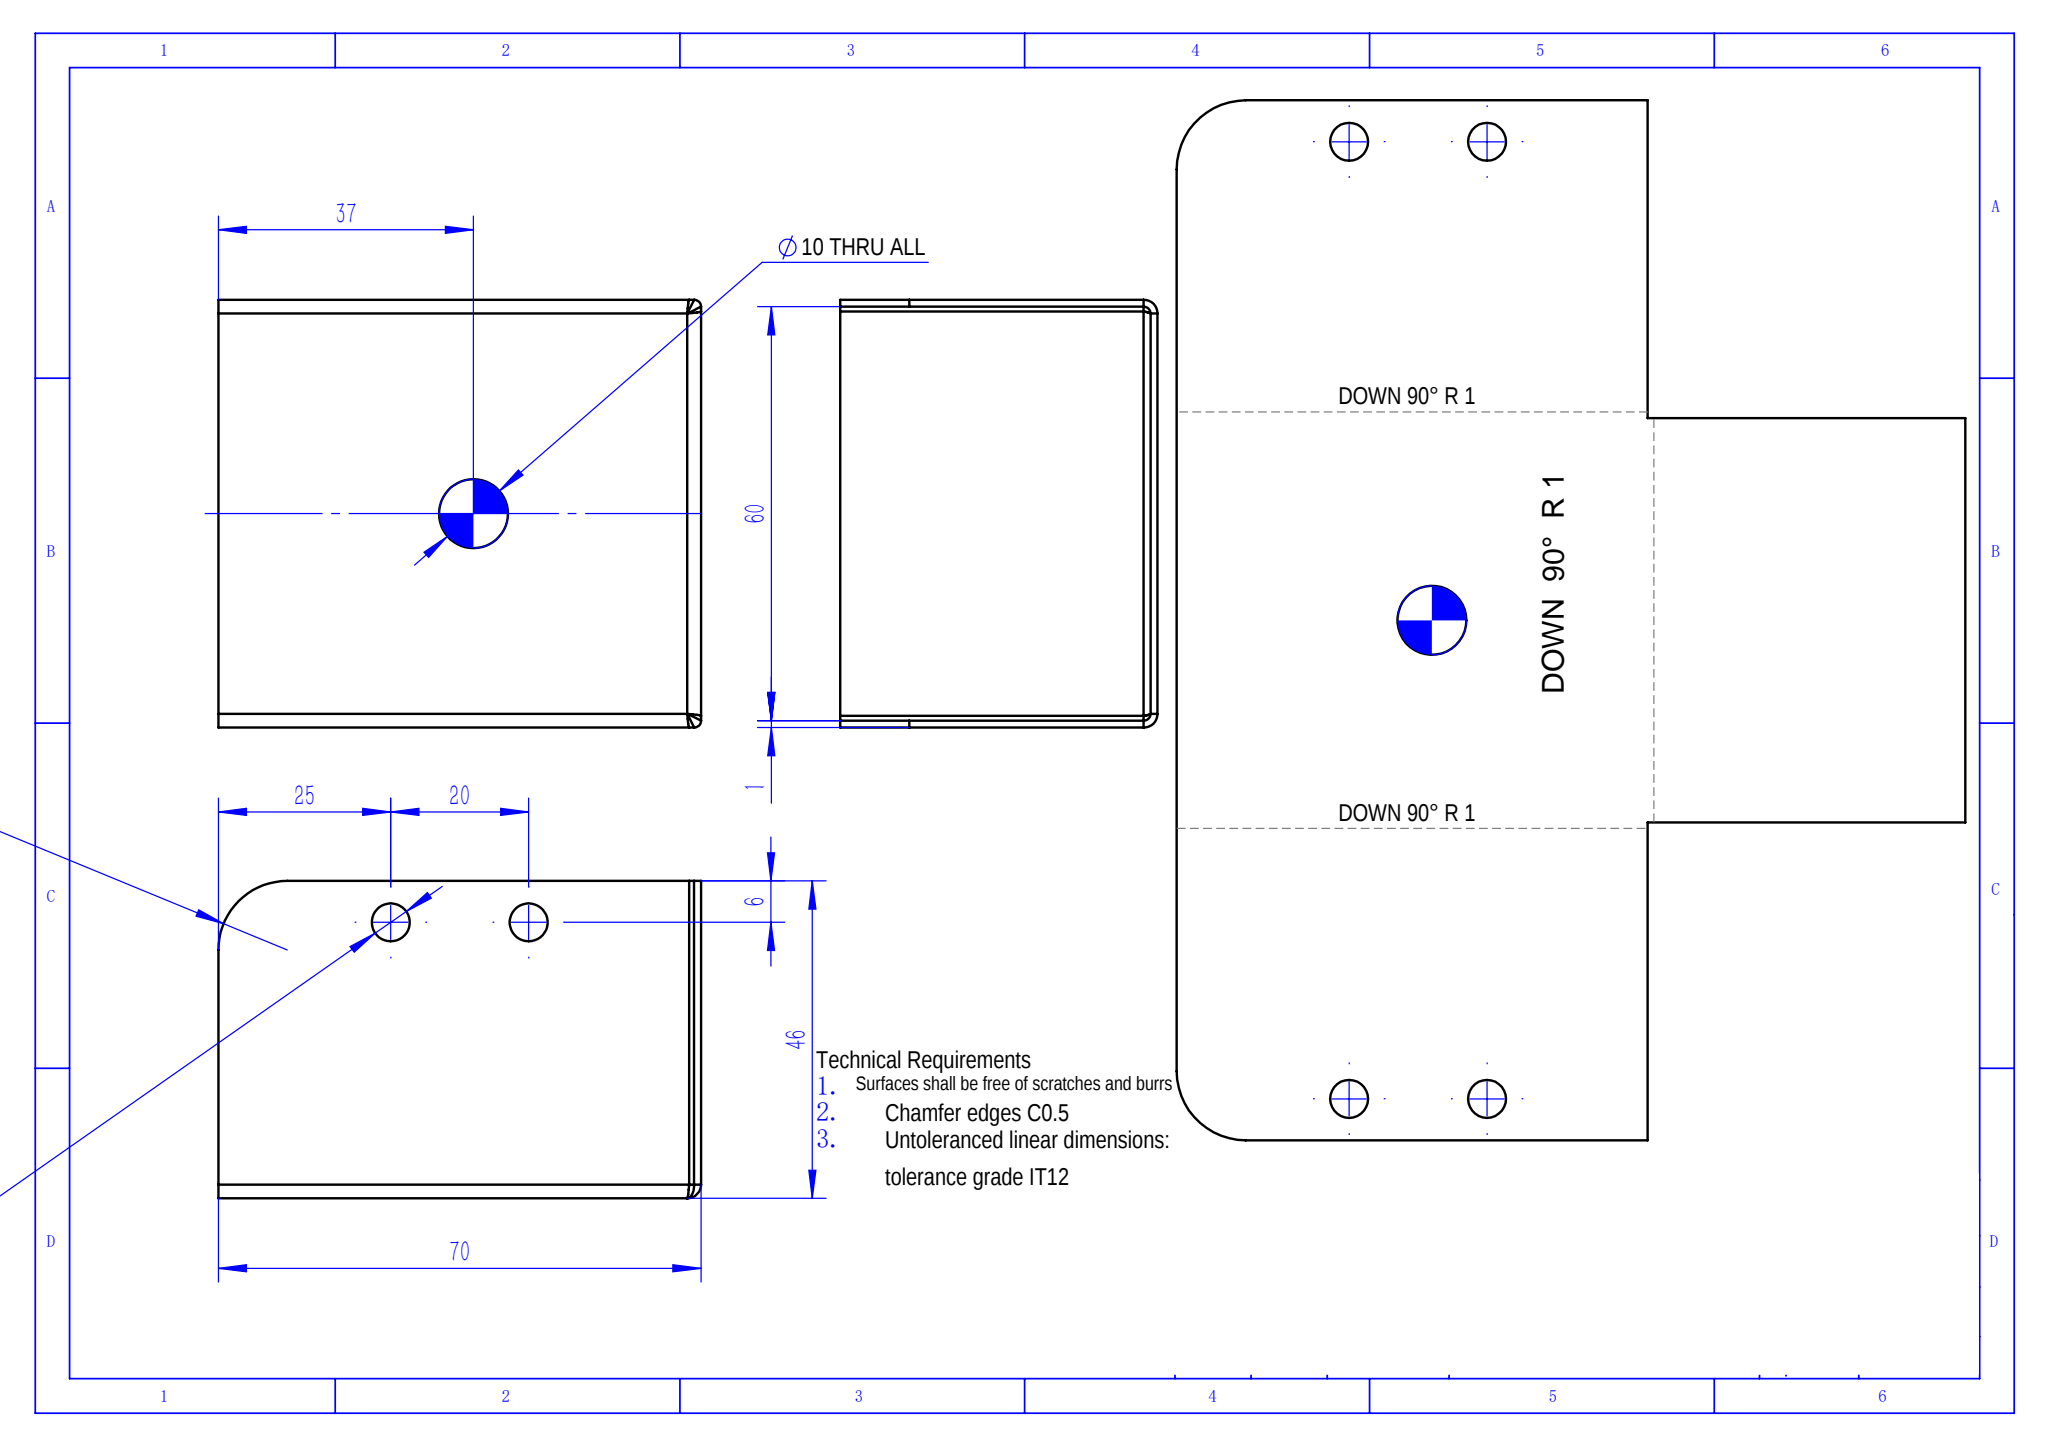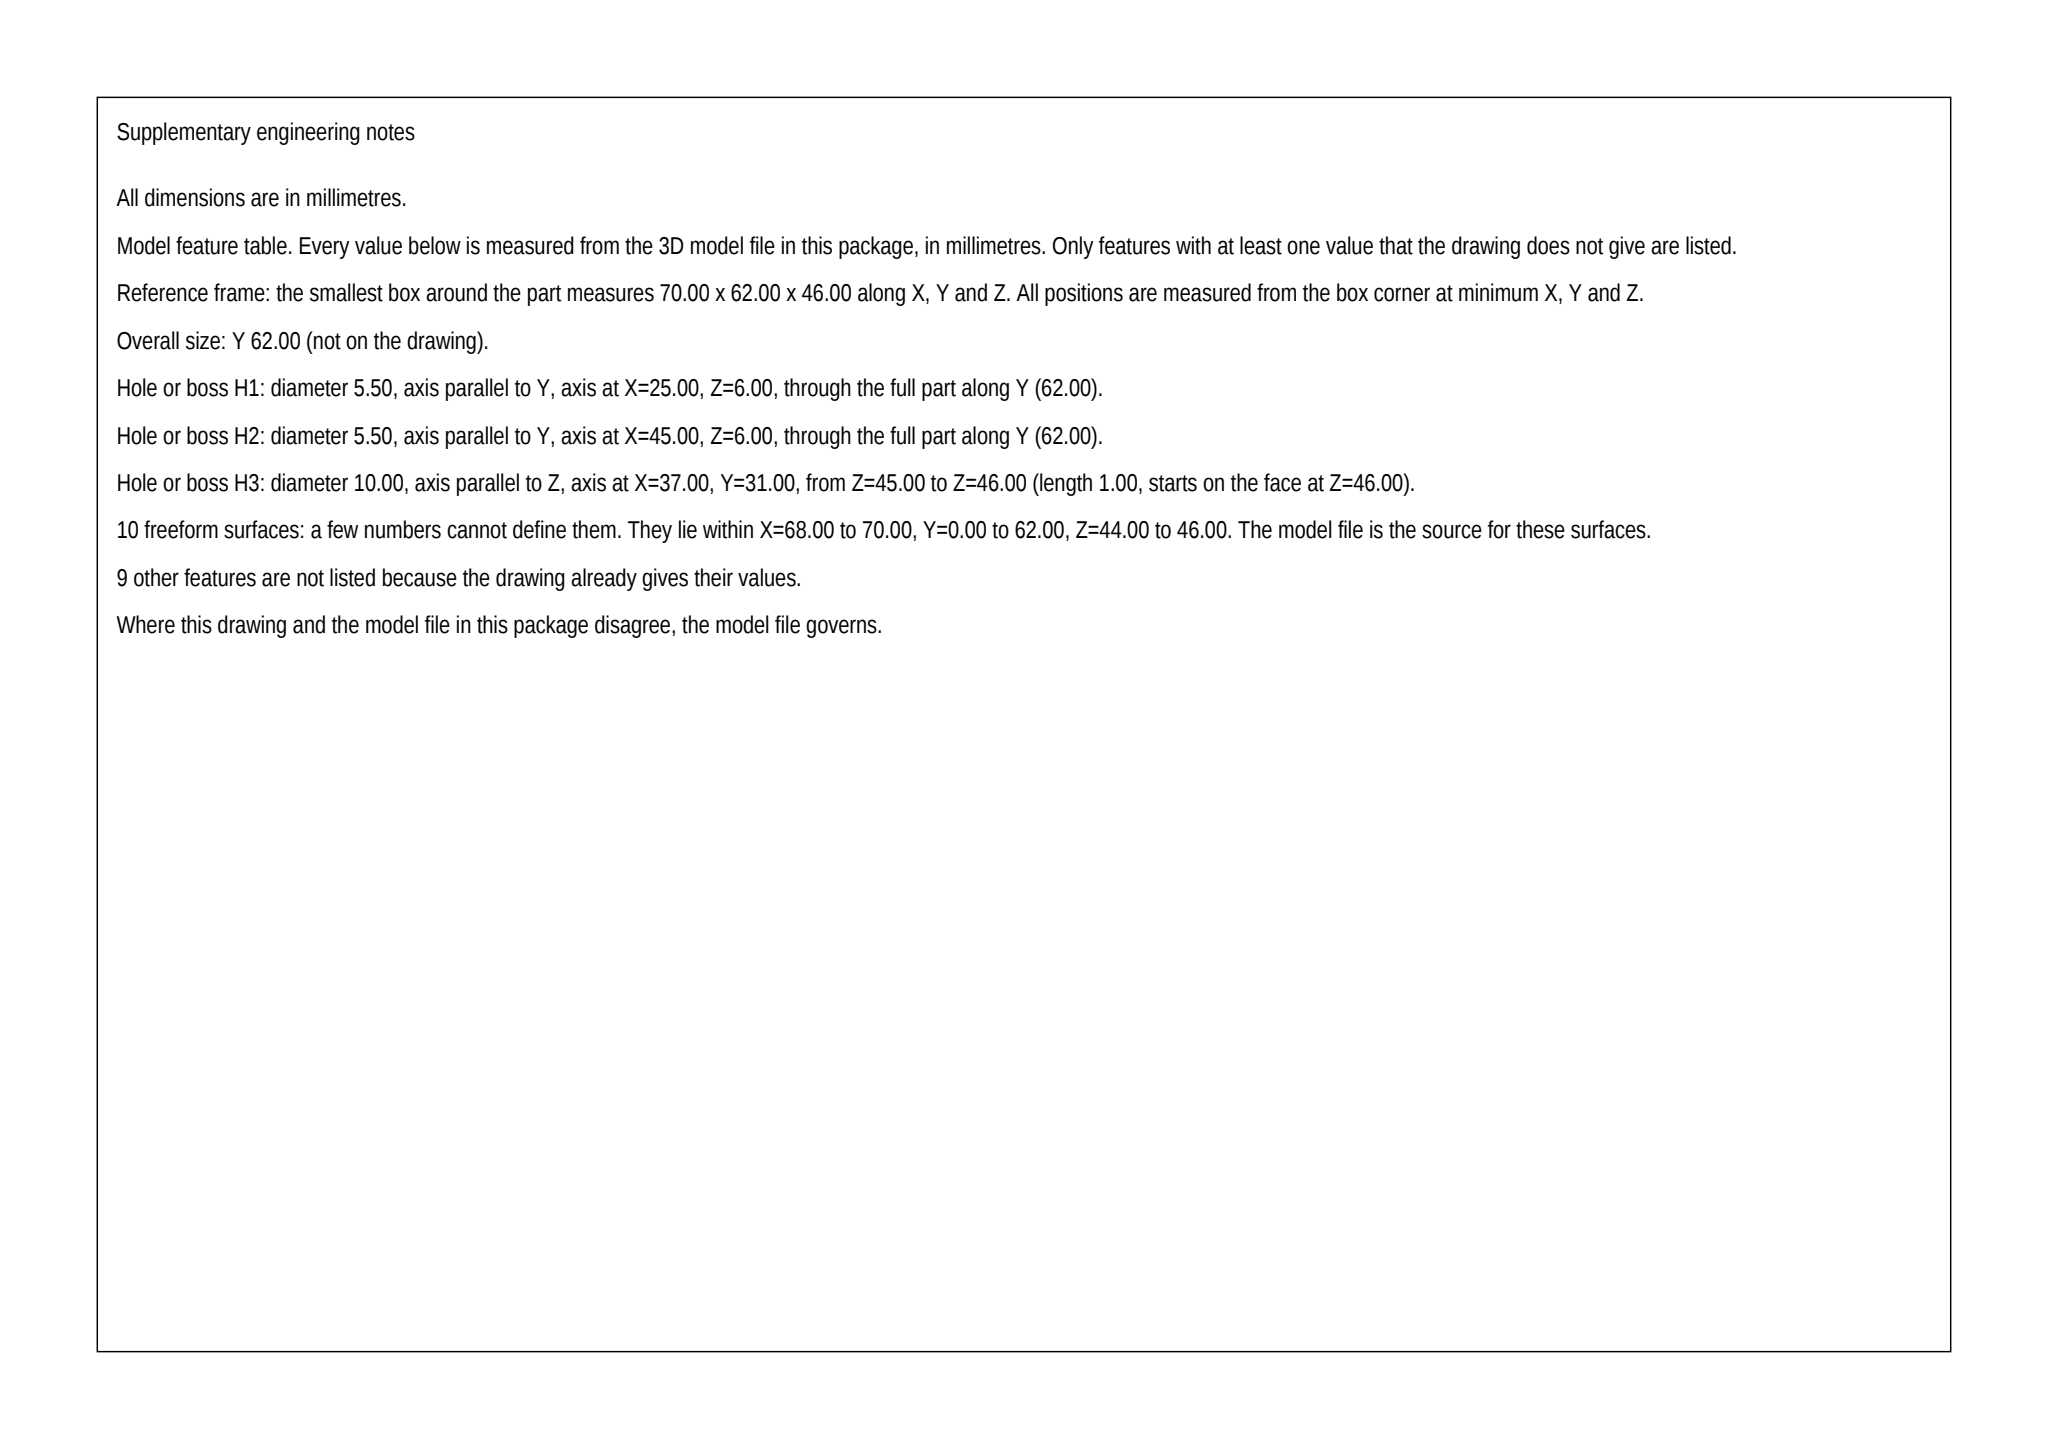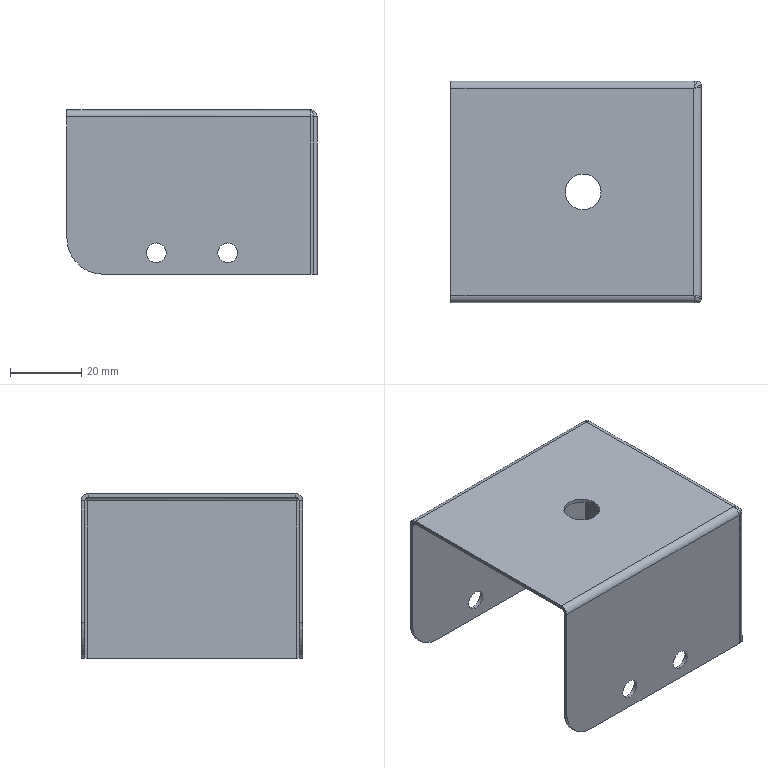Part | SolidWorks | mm | 1 solid | 56 faces | box 70 x 62 x 46 mm | volume 12975 mm3 | plane 26 | cylinder 20 | spline 10 | commonest cylinder face diameters 5.5 x8 2 x5 4 x3 10 x2 20 x2